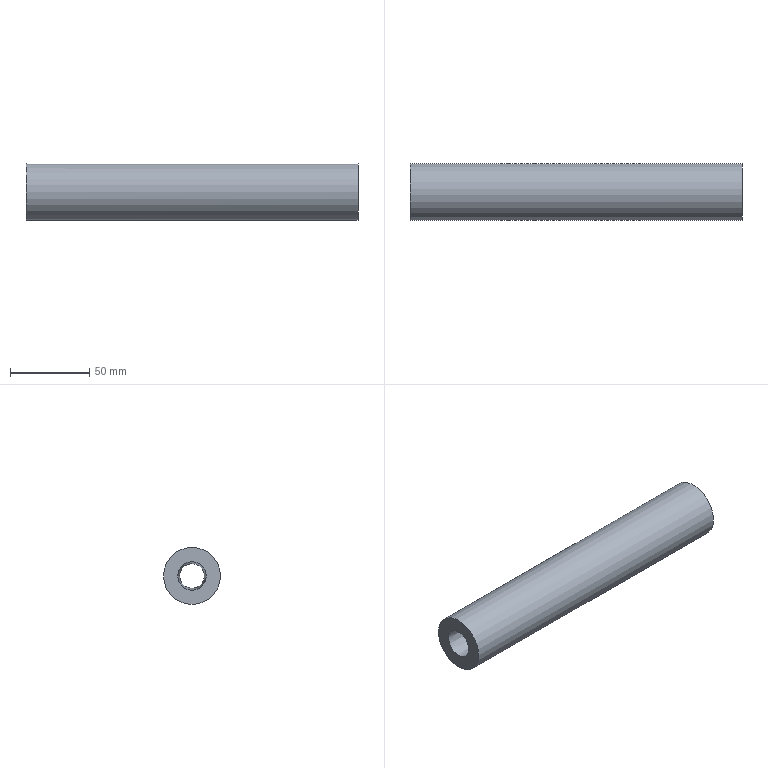Component | NX | SLIDE_SLEEVE | 1 solid | 12 faces | box 210 x 36 x 36 mm | volume 132717 mm3 | plane 8 | cylinder 3 | cone 1 | commonest cylinder face diameters 36 x1 24 x1 20 x1
STEP:
#1=CARTESIAN_POINT('',(0.,0.,0.));
#2=DIRECTION('',(0.,0.,1.));
#3=DIRECTION('',(1.,0.,0.));
#4=AXIS2_PLACEMENT_3D('',#1,#2,#3);
#5=CARTESIAN_POINT('',(152.5,10.,144.));
#6=VERTEX_POINT('',#5);
#7=CARTESIAN_POINT('',(152.5,-10.,144.));
#8=VERTEX_POINT('',#7);
#9=CARTESIAN_POINT('',(152.5,0.,144.));
#10=DIRECTION('',(1.,0.,0.));
#11=DIRECTION('',(0.,1.,0.));
#12=AXIS2_PLACEMENT_3D('',#9,#10,#11);
#13=CIRCLE('',#12,10.);
#14=CARTESIAN_POINT('',(152.5,0.,144.));
#15=DIRECTION('',(1.,0.,0.));
#16=DIRECTION('',(0.,1.,0.));
#17=AXIS2_PLACEMENT_3D('',#14,#15,#16);
#18=PLANE('',#17);
#19=CARTESIAN_POINT('',(0.,0.));
#20=DIRECTION('',(1.,0.));
#21=AXIS2_PLACEMENT_2D('',#19,#20);
#22=CIRCLE('',#21,10.);
#23=(GEOMETRIC_REPRESENTATION_CONTEXT(2)PARAMETRIC_REPRESENTATION_CONTEXT()REPRESENTATION_CONTEXT('',''));
#24=DEFINITIONAL_REPRESENTATION('',(#22),#23);
#25=PCURVE('',#18,#24);
#26=CARTESIAN_POINT('',(190.,0.,144.));
#27=DIRECTION('',(-1.,0.,0.));
#28=DIRECTION('',(0.,-1.,0.));
#29=AXIS2_PLACEMENT_3D('',#26,#27,#28);
#30=CYLINDRICAL_SURFACE('',#29,10.);
#31=CARTESIAN_POINT('',(3.142,37.5));
#32=DIRECTION('',(-1.,0.));
#33=VECTOR('',#32,1.);
#34=LINE('',#31,#33);
#35=(GEOMETRIC_REPRESENTATION_CONTEXT(2)PARAMETRIC_REPRESENTATION_CONTEXT()REPRESENTATION_CONTEXT('',''));
#36=DEFINITIONAL_REPRESENTATION('',(#34),#35);
#37=PCURVE('',#30,#36);
#38=SURFACE_CURVE('',#13,(#25,#37),.PCURVE_S1.);
#39=EDGE_CURVE('',#6,#8,#38,.T.);
#40=ORIENTED_EDGE('',*,*,#39,.T.);
#41=CARTESIAN_POINT('',(152.5,0.,144.));
#42=DIRECTION('',(1.,0.,0.));
#43=DIRECTION('',(0.,1.,0.));
#44=AXIS2_PLACEMENT_3D('',#41,#42,#43);
#45=CIRCLE('',#44,10.);
#46=CARTESIAN_POINT('',(0.,0.));
#47=DIRECTION('',(1.,0.));
#48=AXIS2_PLACEMENT_2D('',#46,#47);
#49=CIRCLE('',#48,10.);
#50=(GEOMETRIC_REPRESENTATION_CONTEXT(2)PARAMETRIC_REPRESENTATION_CONTEXT()REPRESENTATION_CONTEXT('',''));
#51=DEFINITIONAL_REPRESENTATION('',(#49),#50);
#52=PCURVE('',#18,#51);
#53=CARTESIAN_POINT('',(9.425,37.5));
#54=DIRECTION('',(-1.,0.));
#55=VECTOR('',#54,1.);
#56=LINE('',#53,#55);
#57=(GEOMETRIC_REPRESENTATION_CONTEXT(2)PARAMETRIC_REPRESENTATION_CONTEXT()REPRESENTATION_CONTEXT('',''));
#58=DEFINITIONAL_REPRESENTATION('',(#56),#57);
#59=PCURVE('',#30,#58);
#60=SURFACE_CURVE('',#45,(#52,#59),.PCURVE_S1.);
#61=EDGE_CURVE('',#8,#6,#60,.T.);
#62=ORIENTED_EDGE('',*,*,#61,.T.);
#63=EDGE_LOOP('',(#40,#62));
#64=FACE_BOUND('',#63,.T.);
#65=CARTESIAN_POINT('',(152.5,12.,144.));
#66=VERTEX_POINT('',#65);
#67=CARTESIAN_POINT('',(152.5,0.,144.));
#68=DIRECTION('',(1.,0.,0.));
#69=DIRECTION('',(0.,1.,0.));
#70=AXIS2_PLACEMENT_3D('',#67,#68,#69);
#71=CIRCLE('',#70,12.);
#72=CARTESIAN_POINT('',(0.,0.));
#73=DIRECTION('',(1.,0.));
#74=AXIS2_PLACEMENT_2D('',#72,#73);
#75=CIRCLE('',#74,12.);
#76=(GEOMETRIC_REPRESENTATION_CONTEXT(2)PARAMETRIC_REPRESENTATION_CONTEXT()REPRESENTATION_CONTEXT('',''));
#77=DEFINITIONAL_REPRESENTATION('',(#75),#76);
#78=PCURVE('',#18,#77);
#79=CARTESIAN_POINT('',(190.,0.,144.));
#80=DIRECTION('',(1.,0.,0.));
#81=DIRECTION('',(0.,1.,0.));
#82=AXIS2_PLACEMENT_3D('',#79,#80,#81);
#83=CYLINDRICAL_SURFACE('',#82,12.);
#84=CARTESIAN_POINT('',(0.,-37.5));
#85=DIRECTION('',(1.,0.));
#86=VECTOR('',#85,1.);
#87=LINE('',#84,#86);
#88=(GEOMETRIC_REPRESENTATION_CONTEXT(2)PARAMETRIC_REPRESENTATION_CONTEXT()REPRESENTATION_CONTEXT('',''));
#89=DEFINITIONAL_REPRESENTATION('',(#87),#88);
#90=PCURVE('',#83,#89);
#91=SURFACE_CURVE('',#71,(#78,#90),.PCURVE_S1.);
#92=EDGE_CURVE('',#66,#66,#91,.T.);
#93=ORIENTED_EDGE('',*,*,#92,.F.);
#94=EDGE_LOOP('',(#93));
#95=FACE_BOUND('',#94,.T.);
#96=ADVANCED_FACE('',(#64,#95),#18,.F.);
#97=CARTESIAN_POINT('',(190.,2.,126.111));
#98=VERTEX_POINT('',#97);
#99=CARTESIAN_POINT('',(190.,2.,129.));
#100=VERTEX_POINT('',#99);
#101=CARTESIAN_POINT('',(190.,2.,121.5));
#102=DIRECTION('',(0.,-0.,1.));
#103=VECTOR('',#102,1.);
#104=LINE('',#101,#103);
#105=CARTESIAN_POINT('',(190.,0.,144.));
#106=DIRECTION('',(1.,0.,0.));
#107=DIRECTION('',(0.,1.,0.));
#108=AXIS2_PLACEMENT_3D('',#105,#106,#107);
#109=PLANE('',#108);
#110=CARTESIAN_POINT('',(2.,-22.5));
#111=DIRECTION('',(-0.,1.));
#112=VECTOR('',#111,1.);
#113=LINE('',#110,#112);
#114=(GEOMETRIC_REPRESENTATION_CONTEXT(2)PARAMETRIC_REPRESENTATION_CONTEXT()REPRESENTATION_CONTEXT('',''));
#115=DEFINITIONAL_REPRESENTATION('',(#113),#114);
#116=PCURVE('',#109,#115);
#117=CARTESIAN_POINT('',(-2.,2.,121.5));
#118=DIRECTION('',(0.,1.,0.));
#119=DIRECTION('',(0.,-0.,1.));
#120=AXIS2_PLACEMENT_3D('',#117,#118,#119);
#121=PLANE('',#120);
#122=CARTESIAN_POINT('',(0.,192.));
#123=DIRECTION('',(1.,0.));
#124=VECTOR('',#123,1.);
#125=LINE('',#122,#124);
#126=(GEOMETRIC_REPRESENTATION_CONTEXT(2)PARAMETRIC_REPRESENTATION_CONTEXT()REPRESENTATION_CONTEXT('',''));
#127=DEFINITIONAL_REPRESENTATION('',(#125),#126);
#128=PCURVE('',#121,#127);
#129=SURFACE_CURVE('',#104,(#116,#128),.PCURVE_S1.);
#130=EDGE_CURVE('',#98,#100,#129,.T.);
#131=ORIENTED_EDGE('',*,*,#130,.F.);
#132=CARTESIAN_POINT('',(190.,18.,144.));
#133=VERTEX_POINT('',#132);
#134=CARTESIAN_POINT('',(190.,0.,144.));
#135=DIRECTION('',(1.,0.,0.));
#136=DIRECTION('',(0.,1.,0.));
#137=AXIS2_PLACEMENT_3D('',#134,#135,#136);
#138=CIRCLE('',#137,18.);
#139=CARTESIAN_POINT('',(0.,0.));
#140=DIRECTION('',(1.,0.));
#141=AXIS2_PLACEMENT_2D('',#139,#140);
#142=CIRCLE('',#141,18.);
#143=(GEOMETRIC_REPRESENTATION_CONTEXT(2)PARAMETRIC_REPRESENTATION_CONTEXT()REPRESENTATION_CONTEXT('',''));
#144=DEFINITIONAL_REPRESENTATION('',(#142),#143);
#145=PCURVE('',#109,#144);
#146=CARTESIAN_POINT('',(190.,0.,144.));
#147=DIRECTION('',(1.,0.,0.));
#148=DIRECTION('',(0.,1.,0.));
#149=AXIS2_PLACEMENT_3D('',#146,#147,#148);
#150=CYLINDRICAL_SURFACE('',#149,18.);
#151=CARTESIAN_POINT('',(0.,0.));
#152=DIRECTION('',(1.,0.));
#153=VECTOR('',#152,1.);
#154=LINE('',#151,#153);
#155=(GEOMETRIC_REPRESENTATION_CONTEXT(2)PARAMETRIC_REPRESENTATION_CONTEXT()REPRESENTATION_CONTEXT('',''));
#156=DEFINITIONAL_REPRESENTATION('',(#154),#155);
#157=PCURVE('',#150,#156);
#158=SURFACE_CURVE('',#138,(#145,#157),.PCURVE_S1.);
#159=EDGE_CURVE('',#98,#133,#158,.T.);
#160=ORIENTED_EDGE('',*,*,#159,.T.);
#161=CARTESIAN_POINT('',(190.,-2.,126.111));
#162=VERTEX_POINT('',#161);
#163=CARTESIAN_POINT('',(190.,0.,144.));
#164=DIRECTION('',(1.,0.,0.));
#165=DIRECTION('',(0.,1.,0.));
#166=AXIS2_PLACEMENT_3D('',#163,#164,#165);
#167=CIRCLE('',#166,18.);
#168=CARTESIAN_POINT('',(0.,0.));
#169=DIRECTION('',(1.,0.));
#170=AXIS2_PLACEMENT_2D('',#168,#169);
#171=CIRCLE('',#170,18.);
#172=(GEOMETRIC_REPRESENTATION_CONTEXT(2)PARAMETRIC_REPRESENTATION_CONTEXT()REPRESENTATION_CONTEXT('',''));
#173=DEFINITIONAL_REPRESENTATION('',(#171),#172);
#174=PCURVE('',#109,#173);
#175=CARTESIAN_POINT('',(-6.283,0.));
#176=DIRECTION('',(1.,0.));
#177=VECTOR('',#176,1.);
#178=LINE('',#175,#177);
#179=(GEOMETRIC_REPRESENTATION_CONTEXT(2)PARAMETRIC_REPRESENTATION_CONTEXT()REPRESENTATION_CONTEXT('',''));
#180=DEFINITIONAL_REPRESENTATION('',(#178),#179);
#181=PCURVE('',#150,#180);
#182=SURFACE_CURVE('',#167,(#174,#181),.PCURVE_S1.);
#183=EDGE_CURVE('',#133,#162,#182,.T.);
#184=ORIENTED_EDGE('',*,*,#183,.T.);
#185=CARTESIAN_POINT('',(190.,-2.,129.));
#186=VERTEX_POINT('',#185);
#187=CARTESIAN_POINT('',(190.,-2.,129.));
#188=DIRECTION('',(0.,-0.,-1.));
#189=VECTOR('',#188,1.);
#190=LINE('',#187,#189);
#191=CARTESIAN_POINT('',(-2.,-15.));
#192=DIRECTION('',(-0.,-1.));
#193=VECTOR('',#192,1.);
#194=LINE('',#191,#193);
#195=(GEOMETRIC_REPRESENTATION_CONTEXT(2)PARAMETRIC_REPRESENTATION_CONTEXT()REPRESENTATION_CONTEXT('',''));
#196=DEFINITIONAL_REPRESENTATION('',(#194),#195);
#197=PCURVE('',#109,#196);
#198=CARTESIAN_POINT('',(-2.,-2.,129.));
#199=DIRECTION('',(0.,-1.,0.));
#200=DIRECTION('',(0.,-0.,-1.));
#201=AXIS2_PLACEMENT_3D('',#198,#199,#200);
#202=PLANE('',#201);
#203=CARTESIAN_POINT('',(0.,192.));
#204=DIRECTION('',(1.,0.));
#205=VECTOR('',#204,1.);
#206=LINE('',#203,#205);
#207=(GEOMETRIC_REPRESENTATION_CONTEXT(2)PARAMETRIC_REPRESENTATION_CONTEXT()REPRESENTATION_CONTEXT('',''));
#208=DEFINITIONAL_REPRESENTATION('',(#206),#207);
#209=PCURVE('',#202,#208);
#210=SURFACE_CURVE('',#190,(#197,#209),.PCURVE_S1.);
#211=EDGE_CURVE('',#186,#162,#210,.T.);
#212=ORIENTED_EDGE('',*,*,#211,.F.);
#213=CARTESIAN_POINT('',(190.,2.,129.));
#214=DIRECTION('',(0.,-1.,0.));
#215=VECTOR('',#214,1.);
#216=LINE('',#213,#215);
#217=CARTESIAN_POINT('',(2.,-15.));
#218=DIRECTION('',(-1.,0.));
#219=VECTOR('',#218,1.);
#220=LINE('',#217,#219);
#221=(GEOMETRIC_REPRESENTATION_CONTEXT(2)PARAMETRIC_REPRESENTATION_CONTEXT()REPRESENTATION_CONTEXT('',''));
#222=DEFINITIONAL_REPRESENTATION('',(#220),#221);
#223=PCURVE('',#109,#222);
#224=CARTESIAN_POINT('',(-2.,2.,129.));
#225=DIRECTION('',(0.,0.,1.));
#226=DIRECTION('',(0.,-1.,0.));
#227=AXIS2_PLACEMENT_3D('',#224,#225,#226);
#228=PLANE('',#227);
#229=CARTESIAN_POINT('',(0.,192.));
#230=DIRECTION('',(1.,0.));
#231=VECTOR('',#230,1.);
#232=LINE('',#229,#231);
#233=(GEOMETRIC_REPRESENTATION_CONTEXT(2)PARAMETRIC_REPRESENTATION_CONTEXT()REPRESENTATION_CONTEXT('',''));
#234=DEFINITIONAL_REPRESENTATION('',(#232),#233);
#235=PCURVE('',#228,#234);
#236=SURFACE_CURVE('',#216,(#223,#235),.PCURVE_S1.);
#237=EDGE_CURVE('',#100,#186,#236,.T.);
#238=ORIENTED_EDGE('',*,*,#237,.F.);
#239=EDGE_LOOP('',(#131,#160,#184,#212,#238));
#240=FACE_BOUND('',#239,.T.);
#241=CARTESIAN_POINT('',(190.,-10.,144.));
#242=VERTEX_POINT('',#241);
#243=CARTESIAN_POINT('',(190.,0.,144.));
#244=DIRECTION('',(-1.,0.,0.));
#245=DIRECTION('',(0.,-1.,0.));
#246=AXIS2_PLACEMENT_3D('',#243,#244,#245);
#247=CIRCLE('',#246,10.);
#248=CARTESIAN_POINT('',(-10.,0.));
#249=CARTESIAN_POINT('',(-10.,17.321));
#250=CARTESIAN_POINT('',(5.,8.66));
#251=CARTESIAN_POINT('',(20.,0.));
#252=CARTESIAN_POINT('',(5.,-8.66));
#253=CARTESIAN_POINT('',(-10.,-17.321));
#254=CARTESIAN_POINT('',(-10.,0.));
#255=(BOUNDED_CURVE()B_SPLINE_CURVE(2,(#248,#249,#250,#251,#252,#253,#254),.UNSPECIFIED.,.T.,.F.)B_SPLINE_CURVE_WITH_KNOTS((1,2,2,2,2,1),(-2.094,0.,2.094,4.189,6.283,8.378),.UNSPECIFIED.)CURVE()GEOMETRIC_REPRESENTATION_ITEM()RATIONAL_B_SPLINE_CURVE((1.,0.5,1.,0.5,1.,0.5,1.))REPRESENTATION_ITEM(''));
#256=(GEOMETRIC_REPRESENTATION_CONTEXT(2)PARAMETRIC_REPRESENTATION_CONTEXT()REPRESENTATION_CONTEXT('',''));
#257=DEFINITIONAL_REPRESENTATION('',(#255),#256);
#258=PCURVE('',#109,#257);
#259=CARTESIAN_POINT('',(0.,0.));
#260=DIRECTION('',(1.,0.));
#261=VECTOR('',#260,1.);
#262=LINE('',#259,#261);
#263=(GEOMETRIC_REPRESENTATION_CONTEXT(2)PARAMETRIC_REPRESENTATION_CONTEXT()REPRESENTATION_CONTEXT('',''));
#264=DEFINITIONAL_REPRESENTATION('',(#262),#263);
#265=PCURVE('',#30,#264);
#266=SURFACE_CURVE('',#247,(#258,#265),.PCURVE_S1.);
#267=EDGE_CURVE('',#242,#242,#266,.T.);
#268=ORIENTED_EDGE('',*,*,#267,.T.);
#269=EDGE_LOOP('',(#268));
#270=FACE_BOUND('',#269,.T.);
#271=ADVANCED_FACE('',(#240,#270),#109,.T.);
#272=ORIENTED_EDGE('',*,*,#183,.F.);
#273=CARTESIAN_POINT('',(-20.,18.,144.));
#274=VERTEX_POINT('',#273);
#275=CARTESIAN_POINT('',(-20.,18.,144.));
#276=CARTESIAN_POINT('',(190.,18.,144.));
#277=B_SPLINE_CURVE_WITH_KNOTS('',1,(#275,#276),.UNSPECIFIED.,.F.,.F.,(2,2),(-210.,0.),.PIECEWISE_BEZIER_KNOTS.);
#278=CARTESIAN_POINT('',(0.,0.));
#279=DIRECTION('',(0.,1.));
#280=VECTOR('',#279,1.);
#281=LINE('',#278,#280);
#282=(GEOMETRIC_REPRESENTATION_CONTEXT(2)PARAMETRIC_REPRESENTATION_CONTEXT()REPRESENTATION_CONTEXT('',''));
#283=DEFINITIONAL_REPRESENTATION('',(#281),#282);
#284=PCURVE('',#150,#283);
#285=CARTESIAN_POINT('',(6.283,0.));
#286=DIRECTION('',(0.,1.));
#287=VECTOR('',#286,1.);
#288=LINE('',#285,#287);
#289=(GEOMETRIC_REPRESENTATION_CONTEXT(2)PARAMETRIC_REPRESENTATION_CONTEXT()REPRESENTATION_CONTEXT('',''));
#290=DEFINITIONAL_REPRESENTATION('',(#288),#289);
#291=PCURVE('',#150,#290);
#292=SEAM_CURVE('',#277,(#284,#291),.PCURVE_S1.);
#293=EDGE_CURVE('',#274,#133,#292,.T.);
#294=ORIENTED_EDGE('',*,*,#293,.F.);
#295=CARTESIAN_POINT('',(-20.,0.,144.));
#296=DIRECTION('',(1.,0.,0.));
#297=DIRECTION('',(0.,1.,0.));
#298=AXIS2_PLACEMENT_3D('',#295,#296,#297);
#299=CIRCLE('',#298,18.);
#300=CARTESIAN_POINT('',(0.,-210.));
#301=DIRECTION('',(1.,0.));
#302=VECTOR('',#301,1.);
#303=LINE('',#300,#302);
#304=(GEOMETRIC_REPRESENTATION_CONTEXT(2)PARAMETRIC_REPRESENTATION_CONTEXT()REPRESENTATION_CONTEXT('',''));
#305=DEFINITIONAL_REPRESENTATION('',(#303),#304);
#306=PCURVE('',#150,#305);
#307=CARTESIAN_POINT('',(-20.,-9.,144.));
#308=DIRECTION('',(1.,0.,0.));
#309=DIRECTION('',(0.,1.,0.));
#310=AXIS2_PLACEMENT_3D('',#307,#308,#309);
#311=PLANE('',#310);
#312=CARTESIAN_POINT('',(9.,0.));
#313=DIRECTION('',(1.,0.));
#314=AXIS2_PLACEMENT_2D('',#312,#313);
#315=CIRCLE('',#314,18.);
#316=(GEOMETRIC_REPRESENTATION_CONTEXT(2)PARAMETRIC_REPRESENTATION_CONTEXT()REPRESENTATION_CONTEXT('',''));
#317=DEFINITIONAL_REPRESENTATION('',(#315),#316);
#318=PCURVE('',#311,#317);
#319=SURFACE_CURVE('',#299,(#306,#318),.PCURVE_S1.);
#320=EDGE_CURVE('',#274,#274,#319,.T.);
#321=ORIENTED_EDGE('',*,*,#320,.T.);
#322=ORIENTED_EDGE('',*,*,#293,.T.);
#323=ORIENTED_EDGE('',*,*,#159,.F.);
#324=CARTESIAN_POINT('',(-2.,2.,126.111));
#325=VERTEX_POINT('',#324);
#326=CARTESIAN_POINT('',(190.,2.,126.111));
#327=DIRECTION('',(-1.,0.,0.));
#328=VECTOR('',#327,1.);
#329=LINE('',#326,#328);
#330=CARTESIAN_POINT('',(4.824,0.));
#331=DIRECTION('',(0.,-1.));
#332=VECTOR('',#331,1.);
#333=LINE('',#330,#332);
#334=(GEOMETRIC_REPRESENTATION_CONTEXT(2)PARAMETRIC_REPRESENTATION_CONTEXT()REPRESENTATION_CONTEXT('',''));
#335=DEFINITIONAL_REPRESENTATION('',(#333),#334);
#336=PCURVE('',#150,#335);
#337=CARTESIAN_POINT('',(4.611,192.));
#338=DIRECTION('',(0.,-1.));
#339=VECTOR('',#338,1.);
#340=LINE('',#337,#339);
#341=(GEOMETRIC_REPRESENTATION_CONTEXT(2)PARAMETRIC_REPRESENTATION_CONTEXT()REPRESENTATION_CONTEXT('',''));
#342=DEFINITIONAL_REPRESENTATION('',(#340),#341);
#343=PCURVE('',#121,#342);
#344=SURFACE_CURVE('',#329,(#336,#343),.PCURVE_S1.);
#345=EDGE_CURVE('',#98,#325,#344,.T.);
#346=ORIENTED_EDGE('',*,*,#345,.T.);
#347=CARTESIAN_POINT('',(-2.,-2.,126.111));
#348=VERTEX_POINT('',#347);
#349=CARTESIAN_POINT('',(-2.,0.,144.));
#350=DIRECTION('',(1.,0.,0.));
#351=DIRECTION('',(0.,1.,0.));
#352=AXIS2_PLACEMENT_3D('',#349,#350,#351);
#353=CIRCLE('',#352,18.);
#354=CARTESIAN_POINT('',(0.,-192.));
#355=DIRECTION('',(1.,0.));
#356=VECTOR('',#355,1.);
#357=LINE('',#354,#356);
#358=(GEOMETRIC_REPRESENTATION_CONTEXT(2)PARAMETRIC_REPRESENTATION_CONTEXT()REPRESENTATION_CONTEXT('',''));
#359=DEFINITIONAL_REPRESENTATION('',(#357),#358);
#360=PCURVE('',#150,#359);
#361=CARTESIAN_POINT('',(-2.,0.,144.));
#362=DIRECTION('',(1.,0.,0.));
#363=DIRECTION('',(0.,1.,0.));
#364=AXIS2_PLACEMENT_3D('',#361,#362,#363);
#365=PLANE('',#364);
#366=CARTESIAN_POINT('',(0.,0.));
#367=DIRECTION('',(1.,0.));
#368=AXIS2_PLACEMENT_2D('',#366,#367);
#369=CIRCLE('',#368,18.);
#370=(GEOMETRIC_REPRESENTATION_CONTEXT(2)PARAMETRIC_REPRESENTATION_CONTEXT()REPRESENTATION_CONTEXT('',''));
#371=DEFINITIONAL_REPRESENTATION('',(#369),#370);
#372=PCURVE('',#365,#371);
#373=SURFACE_CURVE('',#353,(#360,#372),.PCURVE_S1.);
#374=EDGE_CURVE('',#348,#325,#373,.T.);
#375=ORIENTED_EDGE('',*,*,#374,.F.);
#376=CARTESIAN_POINT('',(190.,-2.,126.111));
#377=DIRECTION('',(1.,0.,0.));
#378=VECTOR('',#377,1.);
#379=LINE('',#376,#378);
#380=CARTESIAN_POINT('',(4.601,0.));
#381=DIRECTION('',(0.,1.));
#382=VECTOR('',#381,1.);
#383=LINE('',#380,#382);
#384=(GEOMETRIC_REPRESENTATION_CONTEXT(2)PARAMETRIC_REPRESENTATION_CONTEXT()REPRESENTATION_CONTEXT('',''));
#385=DEFINITIONAL_REPRESENTATION('',(#383),#384);
#386=PCURVE('',#150,#385);
#387=CARTESIAN_POINT('',(2.889,192.));
#388=DIRECTION('',(0.,1.));
#389=VECTOR('',#388,1.);
#390=LINE('',#387,#389);
#391=(GEOMETRIC_REPRESENTATION_CONTEXT(2)PARAMETRIC_REPRESENTATION_CONTEXT()REPRESENTATION_CONTEXT('',''));
#392=DEFINITIONAL_REPRESENTATION('',(#390),#391);
#393=PCURVE('',#202,#392);
#394=SURFACE_CURVE('',#379,(#386,#393),.PCURVE_S1.);
#395=EDGE_CURVE('',#348,#162,#394,.T.);
#396=ORIENTED_EDGE('',*,*,#395,.T.);
#397=EDGE_LOOP('',(#272,#294,#321,#322,#323,#346,#375,#396));
#398=FACE_BOUND('',#397,.T.);
#399=ADVANCED_FACE('',(#398),#150,.T.);
#400=ORIENTED_EDGE('',*,*,#320,.F.);
#401=EDGE_LOOP('',(#400));
#402=FACE_BOUND('',#401,.T.);
#403=CARTESIAN_POINT('',(-20.,9.,144.));
#404=VERTEX_POINT('',#403);
#405=CARTESIAN_POINT('',(-20.,0.,144.));
#406=DIRECTION('',(1.,0.,0.));
#407=DIRECTION('',(0.,1.,0.));
#408=AXIS2_PLACEMENT_3D('',#405,#406,#407);
#409=CIRCLE('',#408,9.);
#410=CARTESIAN_POINT('',(9.,0.));
#411=DIRECTION('',(1.,0.));
#412=AXIS2_PLACEMENT_2D('',#410,#411);
#413=CIRCLE('',#412,9.);
#414=(GEOMETRIC_REPRESENTATION_CONTEXT(2)PARAMETRIC_REPRESENTATION_CONTEXT()REPRESENTATION_CONTEXT('',''));
#415=DEFINITIONAL_REPRESENTATION('',(#413),#414);
#416=PCURVE('',#311,#415);
#417=CARTESIAN_POINT('',(28.,0.,144.));
#418=DIRECTION('',(-1.,0.,0.));
#419=DIRECTION('',(0.,-1.,0.));
#420=AXIS2_PLACEMENT_3D('',#417,#418,#419);
#421=CONICAL_SURFACE('',#420,7.8,0.02499);
#422=CARTESIAN_POINT('',(9.425,48.));
#423=DIRECTION('',(-1.,0.));
#424=VECTOR('',#423,1.);
#425=LINE('',#422,#424);
#426=(GEOMETRIC_REPRESENTATION_CONTEXT(2)PARAMETRIC_REPRESENTATION_CONTEXT()REPRESENTATION_CONTEXT('',''));
#427=DEFINITIONAL_REPRESENTATION('',(#425),#426);
#428=PCURVE('',#421,#427);
#429=SURFACE_CURVE('',#409,(#416,#428),.PCURVE_S1.);
#430=EDGE_CURVE('',#404,#404,#429,.T.);
#431=ORIENTED_EDGE('',*,*,#430,.T.);
#432=EDGE_LOOP('',(#431));
#433=FACE_BOUND('',#432,.T.);
#434=ADVANCED_FACE('',(#402,#433),#311,.F.);
#435=ORIENTED_EDGE('',*,*,#430,.T.);
#436=CARTESIAN_POINT('',(28.,7.8,144.));
#437=VERTEX_POINT('',#436);
#438=CARTESIAN_POINT('',(28.,7.8,144.));
#439=CARTESIAN_POINT('',(-20.,9.,144.));
#440=B_SPLINE_CURVE_WITH_KNOTS('',1,(#438,#439),.UNSPECIFIED.,.F.,.F.,(2,2),(0.,48.015),.PIECEWISE_BEZIER_KNOTS.);
#441=CARTESIAN_POINT('',(3.142,0.));
#442=DIRECTION('',(0.,1.));
#443=VECTOR('',#442,1.);
#444=LINE('',#441,#443);
#445=(GEOMETRIC_REPRESENTATION_CONTEXT(2)PARAMETRIC_REPRESENTATION_CONTEXT()REPRESENTATION_CONTEXT('',''));
#446=DEFINITIONAL_REPRESENTATION('',(#444),#445);
#447=PCURVE('',#421,#446);
#448=CARTESIAN_POINT('',(9.425,0.));
#449=DIRECTION('',(0.,1.));
#450=VECTOR('',#449,1.);
#451=LINE('',#448,#450);
#452=(GEOMETRIC_REPRESENTATION_CONTEXT(2)PARAMETRIC_REPRESENTATION_CONTEXT()REPRESENTATION_CONTEXT('',''));
#453=DEFINITIONAL_REPRESENTATION('',(#451),#452);
#454=PCURVE('',#421,#453);
#455=SEAM_CURVE('',#440,(#447,#454),.PCURVE_S1.);
#456=EDGE_CURVE('',#437,#404,#455,.T.);
#457=ORIENTED_EDGE('',*,*,#456,.F.);
#458=CARTESIAN_POINT('',(28.,0.,144.));
#459=DIRECTION('',(1.,0.,0.));
#460=DIRECTION('',(0.,1.,0.));
#461=AXIS2_PLACEMENT_3D('',#458,#459,#460);
#462=CIRCLE('',#461,7.8);
#463=CARTESIAN_POINT('',(9.425,0.));
#464=DIRECTION('',(-1.,0.));
#465=VECTOR('',#464,1.);
#466=LINE('',#463,#465);
#467=(GEOMETRIC_REPRESENTATION_CONTEXT(2)PARAMETRIC_REPRESENTATION_CONTEXT()REPRESENTATION_CONTEXT('',''));
#468=DEFINITIONAL_REPRESENTATION('',(#466),#467);
#469=PCURVE('',#421,#468);
#470=CARTESIAN_POINT('',(28.,-12.,144.));
#471=DIRECTION('',(-1.,0.,0.));
#472=DIRECTION('',(0.,-1.,0.));
#473=AXIS2_PLACEMENT_3D('',#470,#471,#472);
#474=PLANE('',#473);
#475=CARTESIAN_POINT('',(-19.8,0.));
#476=CARTESIAN_POINT('',(-19.8,13.51));
#477=CARTESIAN_POINT('',(-8.1,6.755));
#478=CARTESIAN_POINT('',(3.6,0.));
#479=CARTESIAN_POINT('',(-8.1,-6.755));
#480=CARTESIAN_POINT('',(-19.8,-13.51));
#481=CARTESIAN_POINT('',(-19.8,0.));
#482=(BOUNDED_CURVE()B_SPLINE_CURVE(2,(#475,#476,#477,#478,#479,#480,#481),.UNSPECIFIED.,.T.,.F.)B_SPLINE_CURVE_WITH_KNOTS((1,2,2,2,2,1),(-2.094,0.,2.094,4.189,6.283,8.378),.UNSPECIFIED.)CURVE()GEOMETRIC_REPRESENTATION_ITEM()RATIONAL_B_SPLINE_CURVE((1.,0.5,1.,0.5,1.,0.5,1.))REPRESENTATION_ITEM(''));
#483=(GEOMETRIC_REPRESENTATION_CONTEXT(2)PARAMETRIC_REPRESENTATION_CONTEXT()REPRESENTATION_CONTEXT('',''));
#484=DEFINITIONAL_REPRESENTATION('',(#482),#483);
#485=PCURVE('',#474,#484);
#486=SURFACE_CURVE('',#462,(#469,#485),.PCURVE_S1.);
#487=EDGE_CURVE('',#437,#437,#486,.T.);
#488=ORIENTED_EDGE('',*,*,#487,.F.);
#489=ORIENTED_EDGE('',*,*,#456,.T.);
#490=EDGE_LOOP('',(#435,#457,#488,#489));
#491=FACE_BOUND('',#490,.F.);
#492=ADVANCED_FACE('',(#491),#421,.F.);
#493=ORIENTED_EDGE('',*,*,#487,.F.);
#494=EDGE_LOOP('',(#493));
#495=FACE_BOUND('',#494,.T.);
#496=CARTESIAN_POINT('',(28.,12.,144.));
#497=VERTEX_POINT('',#496);
#498=CARTESIAN_POINT('',(28.,0.,144.));
#499=DIRECTION('',(1.,0.,0.));
#500=DIRECTION('',(0.,1.,0.));
#501=AXIS2_PLACEMENT_3D('',#498,#499,#500);
#502=CIRCLE('',#501,12.);
#503=CARTESIAN_POINT('',(-24.,0.));
#504=CARTESIAN_POINT('',(-24.,20.785));
#505=CARTESIAN_POINT('',(-6.,10.392));
#506=CARTESIAN_POINT('',(12.,0.));
#507=CARTESIAN_POINT('',(-6.,-10.392));
#508=CARTESIAN_POINT('',(-24.,-20.785));
#509=CARTESIAN_POINT('',(-24.,0.));
#510=(BOUNDED_CURVE()B_SPLINE_CURVE(2,(#503,#504,#505,#506,#507,#508,#509),.UNSPECIFIED.,.T.,.F.)B_SPLINE_CURVE_WITH_KNOTS((1,2,2,2,2,1),(-2.094,0.,2.094,4.189,6.283,8.378),.UNSPECIFIED.)CURVE()GEOMETRIC_REPRESENTATION_ITEM()RATIONAL_B_SPLINE_CURVE((1.,0.5,1.,0.5,1.,0.5,1.))REPRESENTATION_ITEM(''));
#511=(GEOMETRIC_REPRESENTATION_CONTEXT(2)PARAMETRIC_REPRESENTATION_CONTEXT()REPRESENTATION_CONTEXT('',''));
#512=DEFINITIONAL_REPRESENTATION('',(#510),#511);
#513=PCURVE('',#474,#512);
#514=CARTESIAN_POINT('',(0.,-162.));
#515=DIRECTION('',(1.,0.));
#516=VECTOR('',#515,1.);
#517=LINE('',#514,#516);
#518=(GEOMETRIC_REPRESENTATION_CONTEXT(2)PARAMETRIC_REPRESENTATION_CONTEXT()REPRESENTATION_CONTEXT('',''));
#519=DEFINITIONAL_REPRESENTATION('',(#517),#518);
#520=PCURVE('',#83,#519);
#521=SURFACE_CURVE('',#502,(#513,#520),.PCURVE_S1.);
#522=EDGE_CURVE('',#497,#497,#521,.T.);
#523=ORIENTED_EDGE('',*,*,#522,.T.);
#524=EDGE_LOOP('',(#523));
#525=FACE_BOUND('',#524,.T.);
#526=ADVANCED_FACE('',(#495,#525),#474,.F.);
#527=ORIENTED_EDGE('',*,*,#522,.T.);
#528=CARTESIAN_POINT('',(28.,12.,144.));
#529=CARTESIAN_POINT('',(152.5,12.,144.));
#530=B_SPLINE_CURVE_WITH_KNOTS('',1,(#528,#529),.UNSPECIFIED.,.F.,.F.,(2,2),(-162.,-37.5),.PIECEWISE_BEZIER_KNOTS.);
#531=CARTESIAN_POINT('',(6.283,0.));
#532=DIRECTION('',(0.,1.));
#533=VECTOR('',#532,1.);
#534=LINE('',#531,#533);
#535=(GEOMETRIC_REPRESENTATION_CONTEXT(2)PARAMETRIC_REPRESENTATION_CONTEXT()REPRESENTATION_CONTEXT('',''));
#536=DEFINITIONAL_REPRESENTATION('',(#534),#535);
#537=PCURVE('',#83,#536);
#538=CARTESIAN_POINT('',(0.,0.));
#539=DIRECTION('',(0.,1.));
#540=VECTOR('',#539,1.);
#541=LINE('',#538,#540);
#542=(GEOMETRIC_REPRESENTATION_CONTEXT(2)PARAMETRIC_REPRESENTATION_CONTEXT()REPRESENTATION_CONTEXT('',''));
#543=DEFINITIONAL_REPRESENTATION('',(#541),#542);
#544=PCURVE('',#83,#543);
#545=SEAM_CURVE('',#530,(#537,#544),.PCURVE_S1.);
#546=EDGE_CURVE('',#497,#66,#545,.T.);
#547=ORIENTED_EDGE('',*,*,#546,.T.);
#548=ORIENTED_EDGE('',*,*,#92,.F.);
#549=ORIENTED_EDGE('',*,*,#546,.F.);
#550=EDGE_LOOP('',(#527,#547,#548,#549));
#551=FACE_BOUND('',#550,.F.);
#552=ADVANCED_FACE('',(#551),#83,.F.);
#553=ORIENTED_EDGE('',*,*,#267,.T.);
#554=CARTESIAN_POINT('',(190.,-10.,144.));
#555=CARTESIAN_POINT('',(152.5,-10.,144.));
#556=B_SPLINE_CURVE_WITH_KNOTS('',1,(#554,#555),.UNSPECIFIED.,.F.,.F.,(2,2),(0.,37.5),.PIECEWISE_BEZIER_KNOTS.);
#557=CARTESIAN_POINT('',(6.283,0.));
#558=DIRECTION('',(0.,1.));
#559=VECTOR('',#558,1.);
#560=LINE('',#557,#559);
#561=(GEOMETRIC_REPRESENTATION_CONTEXT(2)PARAMETRIC_REPRESENTATION_CONTEXT()REPRESENTATION_CONTEXT('',''));
#562=DEFINITIONAL_REPRESENTATION('',(#560),#561);
#563=PCURVE('',#30,#562);
#564=CARTESIAN_POINT('',(0.,0.));
#565=DIRECTION('',(0.,1.));
#566=VECTOR('',#565,1.);
#567=LINE('',#564,#566);
#568=(GEOMETRIC_REPRESENTATION_CONTEXT(2)PARAMETRIC_REPRESENTATION_CONTEXT()REPRESENTATION_CONTEXT('',''));
#569=DEFINITIONAL_REPRESENTATION('',(#567),#568);
#570=PCURVE('',#30,#569);
#571=SEAM_CURVE('',#556,(#563,#570),.PCURVE_S1.);
#572=EDGE_CURVE('',#242,#8,#571,.T.);
#573=ORIENTED_EDGE('',*,*,#572,.T.);
#574=ORIENTED_EDGE('',*,*,#61,.T.);
#575=ORIENTED_EDGE('',*,*,#39,.T.);
#576=ORIENTED_EDGE('',*,*,#572,.F.);
#577=EDGE_LOOP('',(#553,#573,#574,#575,#576));
#578=FACE_BOUND('',#577,.F.);
#579=ADVANCED_FACE('',(#578),#30,.F.);
#580=ORIENTED_EDGE('',*,*,#130,.T.);
#581=CARTESIAN_POINT('',(-2.,2.,129.));
#582=VERTEX_POINT('',#581);
#583=CARTESIAN_POINT('',(-2.,2.,129.));
#584=DIRECTION('',(-1.,0.,0.));
#585=VECTOR('',#584,1.);
#586=LINE('',#583,#585);
#587=CARTESIAN_POINT('',(7.5,0.));
#588=DIRECTION('',(0.,-1.));
#589=VECTOR('',#588,1.);
#590=LINE('',#587,#589);
#591=(GEOMETRIC_REPRESENTATION_CONTEXT(2)PARAMETRIC_REPRESENTATION_CONTEXT()REPRESENTATION_CONTEXT('',''));
#592=DEFINITIONAL_REPRESENTATION('',(#590),#591);
#593=PCURVE('',#121,#592);
#594=CARTESIAN_POINT('',(0.,0.));
#595=DIRECTION('',(0.,-1.));
#596=VECTOR('',#595,1.);
#597=LINE('',#594,#596);
#598=(GEOMETRIC_REPRESENTATION_CONTEXT(2)PARAMETRIC_REPRESENTATION_CONTEXT()REPRESENTATION_CONTEXT('',''));
#599=DEFINITIONAL_REPRESENTATION('',(#597),#598);
#600=PCURVE('',#228,#599);
#601=SURFACE_CURVE('',#586,(#593,#600),.PCURVE_S1.);
#602=EDGE_CURVE('',#100,#582,#601,.T.);
#603=ORIENTED_EDGE('',*,*,#602,.T.);
#604=CARTESIAN_POINT('',(-2.,2.,121.5));
#605=DIRECTION('',(0.,0.,-1.));
#606=VECTOR('',#605,1.);
#607=LINE('',#604,#606);
#608=CARTESIAN_POINT('',(0.,0.));
#609=DIRECTION('',(-1.,0.));
#610=VECTOR('',#609,1.);
#611=LINE('',#608,#610);
#612=(GEOMETRIC_REPRESENTATION_CONTEXT(2)PARAMETRIC_REPRESENTATION_CONTEXT()REPRESENTATION_CONTEXT('',''));
#613=DEFINITIONAL_REPRESENTATION('',(#611),#612);
#614=PCURVE('',#121,#613);
#615=CARTESIAN_POINT('',(2.,-22.5));
#616=DIRECTION('',(0.,-1.));
#617=VECTOR('',#616,1.);
#618=LINE('',#615,#617);
#619=(GEOMETRIC_REPRESENTATION_CONTEXT(2)PARAMETRIC_REPRESENTATION_CONTEXT()REPRESENTATION_CONTEXT('',''));
#620=DEFINITIONAL_REPRESENTATION('',(#618),#619);
#621=PCURVE('',#365,#620);
#622=SURFACE_CURVE('',#607,(#614,#621),.PCURVE_S1.);
#623=EDGE_CURVE('',#582,#325,#622,.T.);
#624=ORIENTED_EDGE('',*,*,#623,.T.);
#625=ORIENTED_EDGE('',*,*,#345,.F.);
#626=EDGE_LOOP('',(#580,#603,#624,#625));
#627=FACE_BOUND('',#626,.T.);
#628=ADVANCED_FACE('',(#627),#121,.F.);
#629=CARTESIAN_POINT('',(-2.,-2.,129.));
#630=VERTEX_POINT('',#629);
#631=CARTESIAN_POINT('',(-2.,-2.,129.));
#632=DIRECTION('',(0.,0.,1.));
#633=VECTOR('',#632,1.);
#634=LINE('',#631,#633);
#635=CARTESIAN_POINT('',(0.,0.));
#636=DIRECTION('',(-1.,0.));
#637=VECTOR('',#636,1.);
#638=LINE('',#635,#637);
#639=(GEOMETRIC_REPRESENTATION_CONTEXT(2)PARAMETRIC_REPRESENTATION_CONTEXT()REPRESENTATION_CONTEXT('',''));
#640=DEFINITIONAL_REPRESENTATION('',(#638),#639);
#641=PCURVE('',#202,#640);
#642=CARTESIAN_POINT('',(-2.,-15.));
#643=DIRECTION('',(0.,1.));
#644=VECTOR('',#643,1.);
#645=LINE('',#642,#644);
#646=(GEOMETRIC_REPRESENTATION_CONTEXT(2)PARAMETRIC_REPRESENTATION_CONTEXT()REPRESENTATION_CONTEXT('',''));
#647=DEFINITIONAL_REPRESENTATION('',(#645),#646);
#648=PCURVE('',#365,#647);
#649=SURFACE_CURVE('',#634,(#641,#648),.PCURVE_S1.);
#650=EDGE_CURVE('',#348,#630,#649,.T.);
#651=ORIENTED_EDGE('',*,*,#650,.T.);
#652=CARTESIAN_POINT('',(-2.,-2.,129.));
#653=DIRECTION('',(-1.,0.,0.));
#654=VECTOR('',#653,1.);
#655=LINE('',#652,#654);
#656=CARTESIAN_POINT('',(0.,0.));
#657=DIRECTION('',(0.,-1.));
#658=VECTOR('',#657,1.);
#659=LINE('',#656,#658);
#660=(GEOMETRIC_REPRESENTATION_CONTEXT(2)PARAMETRIC_REPRESENTATION_CONTEXT()REPRESENTATION_CONTEXT('',''));
#661=DEFINITIONAL_REPRESENTATION('',(#659),#660);
#662=PCURVE('',#202,#661);
#663=CARTESIAN_POINT('',(4.,0.));
#664=DIRECTION('',(0.,-1.));
#665=VECTOR('',#664,1.);
#666=LINE('',#663,#665);
#667=(GEOMETRIC_REPRESENTATION_CONTEXT(2)PARAMETRIC_REPRESENTATION_CONTEXT()REPRESENTATION_CONTEXT('',''));
#668=DEFINITIONAL_REPRESENTATION('',(#666),#667);
#669=PCURVE('',#228,#668);
#670=SURFACE_CURVE('',#655,(#662,#669),.PCURVE_S1.);
#671=EDGE_CURVE('',#186,#630,#670,.T.);
#672=ORIENTED_EDGE('',*,*,#671,.F.);
#673=ORIENTED_EDGE('',*,*,#211,.T.);
#674=ORIENTED_EDGE('',*,*,#395,.F.);
#675=EDGE_LOOP('',(#651,#672,#673,#674));
#676=FACE_BOUND('',#675,.T.);
#677=ADVANCED_FACE('',(#676),#202,.F.);
#678=ORIENTED_EDGE('',*,*,#374,.T.);
#679=ORIENTED_EDGE('',*,*,#623,.F.);
#680=CARTESIAN_POINT('',(-2.,2.,129.));
#681=DIRECTION('',(0.,1.,0.));
#682=VECTOR('',#681,1.);
#683=LINE('',#680,#682);
#684=CARTESIAN_POINT('',(2.,-15.));
#685=DIRECTION('',(1.,0.));
#686=VECTOR('',#685,1.);
#687=LINE('',#684,#686);
#688=(GEOMETRIC_REPRESENTATION_CONTEXT(2)PARAMETRIC_REPRESENTATION_CONTEXT()REPRESENTATION_CONTEXT('',''));
#689=DEFINITIONAL_REPRESENTATION('',(#687),#688);
#690=PCURVE('',#365,#689);
#691=CARTESIAN_POINT('',(0.,0.));
#692=DIRECTION('',(-1.,0.));
#693=VECTOR('',#692,1.);
#694=LINE('',#691,#693);
#695=(GEOMETRIC_REPRESENTATION_CONTEXT(2)PARAMETRIC_REPRESENTATION_CONTEXT()REPRESENTATION_CONTEXT('',''));
#696=DEFINITIONAL_REPRESENTATION('',(#694),#695);
#697=PCURVE('',#228,#696);
#698=SURFACE_CURVE('',#683,(#690,#697),.PCURVE_S1.);
#699=EDGE_CURVE('',#630,#582,#698,.T.);
#700=ORIENTED_EDGE('',*,*,#699,.F.);
#701=ORIENTED_EDGE('',*,*,#650,.F.);
#702=EDGE_LOOP('',(#678,#679,#700,#701));
#703=FACE_BOUND('',#702,.T.);
#704=ADVANCED_FACE('',(#703),#365,.T.);
#705=ORIENTED_EDGE('',*,*,#237,.T.);
#706=ORIENTED_EDGE('',*,*,#671,.T.);
#707=ORIENTED_EDGE('',*,*,#699,.T.);
#708=ORIENTED_EDGE('',*,*,#602,.F.);
#709=EDGE_LOOP('',(#705,#706,#707,#708));
#710=FACE_BOUND('',#709,.T.);
#711=ADVANCED_FACE('',(#710),#228,.F.);
#712=CLOSED_SHELL('',(#96,#271,#399,#434,#492,#526,#552,#579,#628,#677,#704,#711));
#713=MANIFOLD_SOLID_BREP('',#712);
#714=(LENGTH_UNIT()NAMED_UNIT(*)SI_UNIT(.MILLI.,.METRE.));
#715=UNCERTAINTY_MEASURE_WITH_UNIT(LENGTH_MEASURE(0.000005),#714,'','');
#716=(NAMED_UNIT(*)PLANE_ANGLE_UNIT()SI_UNIT($,.RADIAN.));
#717=(NAMED_UNIT(*)SI_UNIT($,.STERADIAN.)SOLID_ANGLE_UNIT());
#718=(GEOMETRIC_REPRESENTATION_CONTEXT(3)GLOBAL_UNCERTAINTY_ASSIGNED_CONTEXT((#715))GLOBAL_UNIT_ASSIGNED_CONTEXT((#714,#716,#717))REPRESENTATION_CONTEXT('',''));
#719=ADVANCED_BREP_SHAPE_REPRESENTATION('',(#4,#713),#718);